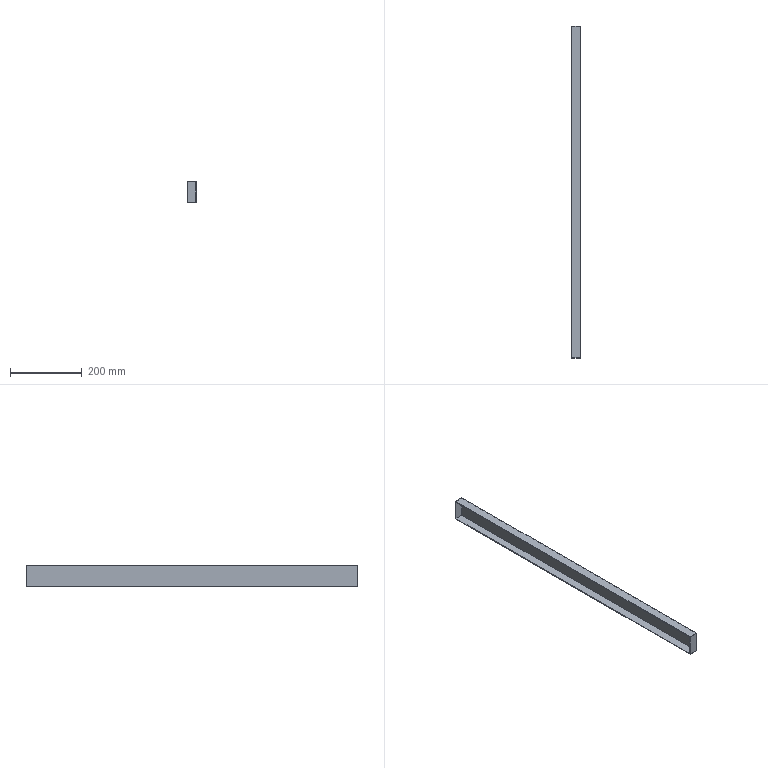Component | SolidWorks | SolderBox-1 | 1 solid | 11 faces | box 25 x 925 x 60 mm | volume 201252 mm3 | plane 11 | material Plain Carbon Steel
build123d program:
from build123d import *

# Parameters (mm, degrees)
SKETCH1_W           = 925
SKETCH1_H           = 60
BOSS_EXTRUDE1_DEPTH = 25
SHELL1_T            = -2


with BuildPart() as part:
    # Sketch1 → Boss-Extrude1 (new body)
    with BuildSketch(Plane.XY):
        Rectangle(SKETCH1_W, SKETCH1_H)
    extrude(amount=BOSS_EXTRUDE1_DEPTH)

    # Shell1
    shell1_openings = [part.faces().sort_by_distance(p)[0] for p in [
        (0, 0, 25),
    ]]
    offset(amount=SHELL1_T, openings=shell1_openings, kind=Kind.INTERSECTION)


solid = part.part

# Placed as in the assembly
solid = solid.moved(Location((-806.135, 72.093, 1073.102), (90, -90, 0)))
STEP:
#1=COLOUR_RGB('',0.7922,0.8196,0.9333);
#2=FILL_AREA_STYLE_COLOUR('',#1);
#3=FILL_AREA_STYLE('',(#2));
#4=SURFACE_STYLE_FILL_AREA(#3);
#5=SURFACE_SIDE_STYLE('',(#4));
#6=SURFACE_STYLE_USAGE(.BOTH.,#5);
#7=PRESENTATION_STYLE_ASSIGNMENT((#6));
#8=CARTESIAN_POINT('',(-31.738,21.047,43.429));
#9=VERTEX_POINT('',#8);
#10=CARTESIAN_POINT('',(-31.738,21.047,41.067));
#11=VERTEX_POINT('',#10);
#12=CARTESIAN_POINT('',(-31.738,21.047,41.067));
#13=DIRECTION('',(-0.,0.,-1.));
#14=VECTOR('',#13,39.37);
#15=LINE('',#12,#14);
#16=EDGE_CURVE('',#9,#11,#15,.T.);
#17=ORIENTED_EDGE('',*,*,#16,.T.);
#18=CARTESIAN_POINT('',(-32.722,21.047,41.067));
#19=VERTEX_POINT('',#18);
#20=CARTESIAN_POINT('',(-32.722,21.047,41.067));
#21=DIRECTION('',(1.,0.,-0.));
#22=VECTOR('',#21,39.37);
#23=LINE('',#20,#22);
#24=EDGE_CURVE('',#19,#11,#23,.T.);
#25=ORIENTED_EDGE('',*,*,#24,.F.);
#26=CARTESIAN_POINT('',(-32.722,21.047,43.429));
#27=VERTEX_POINT('',#26);
#28=CARTESIAN_POINT('',(-32.722,21.047,41.067));
#29=DIRECTION('',(-0.,0.,-1.));
#30=VECTOR('',#29,39.37);
#31=LINE('',#28,#30);
#32=EDGE_CURVE('',#27,#19,#31,.T.);
#33=ORIENTED_EDGE('',*,*,#32,.F.);
#34=CARTESIAN_POINT('',(-32.722,21.047,43.429));
#35=DIRECTION('',(1.,0.,-0.));
#36=VECTOR('',#35,39.37);
#37=LINE('',#34,#36);
#38=EDGE_CURVE('',#27,#9,#37,.T.);
#39=ORIENTED_EDGE('',*,*,#38,.T.);
#40=EDGE_LOOP('',(#17,#25,#33,#39));
#41=FACE_OUTER_BOUND('',#40,.T.);
#42=CARTESIAN_POINT('',(-32.722,21.047,41.067));
#43=DIRECTION('',(0.,-1.,-0.));
#44=DIRECTION('',(1.,0.,-0.));
#45=AXIS2_PLACEMENT_3D('',#42,#43,#44);
#46=PLANE('',#45);
#47=ADVANCED_FACE('',(#41),#46,.F.);
#48=CARTESIAN_POINT('',(-31.738,-15.37,41.067));
#49=VERTEX_POINT('',#48);
#50=CARTESIAN_POINT('',(-31.738,-15.37,41.067));
#51=DIRECTION('',(0.,-1.,0.));
#52=VECTOR('',#51,39.37);
#53=LINE('',#50,#52);
#54=EDGE_CURVE('',#11,#49,#53,.T.);
#55=ORIENTED_EDGE('',*,*,#54,.T.);
#56=CARTESIAN_POINT('',(-32.722,-15.37,41.067));
#57=VERTEX_POINT('',#56);
#58=CARTESIAN_POINT('',(-32.722,-15.37,41.067));
#59=DIRECTION('',(1.,0.,-0.));
#60=VECTOR('',#59,39.37);
#61=LINE('',#58,#60);
#62=EDGE_CURVE('',#57,#49,#61,.T.);
#63=ORIENTED_EDGE('',*,*,#62,.F.);
#64=CARTESIAN_POINT('',(-32.722,-15.37,41.067));
#65=DIRECTION('',(0.,-1.,0.));
#66=VECTOR('',#65,39.37);
#67=LINE('',#64,#66);
#68=EDGE_CURVE('',#19,#57,#67,.T.);
#69=ORIENTED_EDGE('',*,*,#68,.F.);
#70=ORIENTED_EDGE('',*,*,#24,.T.);
#71=EDGE_LOOP('',(#55,#63,#69,#70));
#72=FACE_OUTER_BOUND('',#71,.T.);
#73=CARTESIAN_POINT('',(-32.722,-15.37,41.067));
#74=DIRECTION('',(0.,0.,1.));
#75=DIRECTION('',(-0.,1.,-0.));
#76=AXIS2_PLACEMENT_3D('',#73,#74,#75);
#77=PLANE('',#76);
#78=ADVANCED_FACE('',(#72),#77,.F.);
#79=CARTESIAN_POINT('',(-31.738,-15.37,43.429));
#80=VERTEX_POINT('',#79);
#81=CARTESIAN_POINT('',(-31.738,-15.37,41.067));
#82=DIRECTION('',(0.,-0.,1.));
#83=VECTOR('',#82,39.37);
#84=LINE('',#81,#83);
#85=EDGE_CURVE('',#49,#80,#84,.T.);
#86=ORIENTED_EDGE('',*,*,#85,.T.);
#87=CARTESIAN_POINT('',(-32.722,-15.37,43.429));
#88=VERTEX_POINT('',#87);
#89=CARTESIAN_POINT('',(-32.722,-15.37,43.429));
#90=DIRECTION('',(1.,0.,-0.));
#91=VECTOR('',#90,39.37);
#92=LINE('',#89,#91);
#93=EDGE_CURVE('',#88,#80,#92,.T.);
#94=ORIENTED_EDGE('',*,*,#93,.F.);
#95=CARTESIAN_POINT('',(-32.722,-15.37,41.067));
#96=DIRECTION('',(0.,-0.,1.));
#97=VECTOR('',#96,39.37);
#98=LINE('',#95,#97);
#99=EDGE_CURVE('',#57,#88,#98,.T.);
#100=ORIENTED_EDGE('',*,*,#99,.F.);
#101=ORIENTED_EDGE('',*,*,#62,.T.);
#102=EDGE_LOOP('',(#86,#94,#100,#101));
#103=FACE_OUTER_BOUND('',#102,.T.);
#104=CARTESIAN_POINT('',(-32.722,-15.37,41.067));
#105=DIRECTION('',(-0.,1.,0.));
#106=DIRECTION('',(-1.,-0.,0.));
#107=AXIS2_PLACEMENT_3D('',#104,#105,#106);
#108=PLANE('',#107);
#109=ADVANCED_FACE('',(#103),#108,.F.);
#110=CARTESIAN_POINT('',(-31.738,-15.37,43.429));
#111=DIRECTION('',(-0.,1.,-0.));
#112=VECTOR('',#111,39.37);
#113=LINE('',#110,#112);
#114=EDGE_CURVE('',#80,#9,#113,.T.);
#115=ORIENTED_EDGE('',*,*,#114,.T.);
#116=ORIENTED_EDGE('',*,*,#38,.F.);
#117=CARTESIAN_POINT('',(-32.722,-15.37,43.429));
#118=DIRECTION('',(-0.,1.,-0.));
#119=VECTOR('',#118,39.37);
#120=LINE('',#117,#119);
#121=EDGE_CURVE('',#88,#27,#120,.T.);
#122=ORIENTED_EDGE('',*,*,#121,.F.);
#123=ORIENTED_EDGE('',*,*,#93,.T.);
#124=EDGE_LOOP('',(#115,#116,#122,#123));
#125=FACE_OUTER_BOUND('',#124,.T.);
#126=CARTESIAN_POINT('',(-32.722,-15.37,43.429));
#127=DIRECTION('',(-0.,-0.,-1.));
#128=DIRECTION('',(0.,-1.,0.));
#129=AXIS2_PLACEMENT_3D('',#126,#127,#128);
#130=PLANE('',#129);
#131=ADVANCED_FACE('',(#125),#130,.F.);
#132=CARTESIAN_POINT('',(-32.722,20.968,43.35));
#133=VERTEX_POINT('',#132);
#134=CARTESIAN_POINT('',(-32.722,20.968,41.146));
#135=VERTEX_POINT('',#134);
#136=CARTESIAN_POINT('',(-32.722,20.968,41.067));
#137=DIRECTION('',(-0.,0.,-1.));
#138=VECTOR('',#137,39.37);
#139=LINE('',#136,#138);
#140=EDGE_CURVE('',#133,#135,#139,.T.);
#141=ORIENTED_EDGE('',*,*,#140,.F.);
#142=CARTESIAN_POINT('',(-32.722,-15.292,43.35));
#143=VERTEX_POINT('',#142);
#144=CARTESIAN_POINT('',(-32.722,-15.37,43.35));
#145=DIRECTION('',(-0.,1.,-0.));
#146=VECTOR('',#145,39.37);
#147=LINE('',#144,#146);
#148=EDGE_CURVE('',#143,#133,#147,.T.);
#149=ORIENTED_EDGE('',*,*,#148,.F.);
#150=CARTESIAN_POINT('',(-32.722,-15.292,41.146));
#151=VERTEX_POINT('',#150);
#152=CARTESIAN_POINT('',(-32.722,-15.292,41.067));
#153=DIRECTION('',(0.,-0.,1.));
#154=VECTOR('',#153,39.37);
#155=LINE('',#152,#154);
#156=EDGE_CURVE('',#151,#143,#155,.T.);
#157=ORIENTED_EDGE('',*,*,#156,.F.);
#158=CARTESIAN_POINT('',(-32.722,-15.37,41.146));
#159=DIRECTION('',(0.,-1.,0.));
#160=VECTOR('',#159,39.37);
#161=LINE('',#158,#160);
#162=EDGE_CURVE('',#135,#151,#161,.T.);
#163=ORIENTED_EDGE('',*,*,#162,.F.);
#164=EDGE_LOOP('',(#141,#149,#157,#163));
#165=FACE_BOUND('',#164,.T.);
#166=ORIENTED_EDGE('',*,*,#32,.T.);
#167=ORIENTED_EDGE('',*,*,#68,.T.);
#168=ORIENTED_EDGE('',*,*,#99,.T.);
#169=ORIENTED_EDGE('',*,*,#121,.T.);
#170=EDGE_LOOP('',(#166,#167,#168,#169));
#171=FACE_OUTER_BOUND('',#170,.T.);
#172=CARTESIAN_POINT('',(-32.722,2.838,42.248));
#173=DIRECTION('',(-1.,-0.,0.));
#174=DIRECTION('',(0.,-1.,-0.));
#175=AXIS2_PLACEMENT_3D('',#172,#173,#174);
#176=PLANE('',#175);
#177=ADVANCED_FACE('',(#165,#171),#176,.T.);
#178=ORIENTED_EDGE('',*,*,#16,.F.);
#179=ORIENTED_EDGE('',*,*,#114,.F.);
#180=ORIENTED_EDGE('',*,*,#85,.F.);
#181=ORIENTED_EDGE('',*,*,#54,.F.);
#182=EDGE_LOOP('',(#178,#179,#180,#181));
#183=FACE_OUTER_BOUND('',#182,.T.);
#184=CARTESIAN_POINT('',(-31.738,2.838,42.248));
#185=DIRECTION('',(-1.,-0.,0.));
#186=DIRECTION('',(0.,-1.,-0.));
#187=AXIS2_PLACEMENT_3D('',#184,#185,#186);
#188=PLANE('',#187);
#189=ADVANCED_FACE('',(#183),#188,.F.);
#190=CARTESIAN_POINT('',(-31.816,20.968,43.35));
#191=VERTEX_POINT('',#190);
#192=CARTESIAN_POINT('',(-31.816,20.968,41.146));
#193=VERTEX_POINT('',#192);
#194=CARTESIAN_POINT('',(-31.816,20.968,41.067));
#195=DIRECTION('',(-0.,0.,-1.));
#196=VECTOR('',#195,39.37);
#197=LINE('',#194,#196);
#198=EDGE_CURVE('',#191,#193,#197,.T.);
#199=ORIENTED_EDGE('',*,*,#198,.F.);
#200=CARTESIAN_POINT('',(-32.722,20.968,43.35));
#201=DIRECTION('',(1.,0.,-0.));
#202=VECTOR('',#201,39.37);
#203=LINE('',#200,#202);
#204=EDGE_CURVE('',#133,#191,#203,.T.);
#205=ORIENTED_EDGE('',*,*,#204,.F.);
#206=ORIENTED_EDGE('',*,*,#140,.T.);
#207=CARTESIAN_POINT('',(-32.722,20.968,41.146));
#208=DIRECTION('',(1.,0.,-0.));
#209=VECTOR('',#208,39.37);
#210=LINE('',#207,#209);
#211=EDGE_CURVE('',#135,#193,#210,.T.);
#212=ORIENTED_EDGE('',*,*,#211,.T.);
#213=EDGE_LOOP('',(#199,#205,#206,#212));
#214=FACE_OUTER_BOUND('',#213,.T.);
#215=CARTESIAN_POINT('',(-32.722,20.968,41.067));
#216=DIRECTION('',(0.,-1.,-0.));
#217=DIRECTION('',(1.,0.,-0.));
#218=AXIS2_PLACEMENT_3D('',#215,#216,#217);
#219=PLANE('',#218);
#220=ADVANCED_FACE('',(#214),#219,.T.);
#221=CARTESIAN_POINT('',(-31.816,-15.292,41.146));
#222=VERTEX_POINT('',#221);
#223=CARTESIAN_POINT('',(-31.816,-15.37,41.146));
#224=DIRECTION('',(0.,-1.,0.));
#225=VECTOR('',#224,39.37);
#226=LINE('',#223,#225);
#227=EDGE_CURVE('',#193,#222,#226,.T.);
#228=ORIENTED_EDGE('',*,*,#227,.F.);
#229=ORIENTED_EDGE('',*,*,#211,.F.);
#230=ORIENTED_EDGE('',*,*,#162,.T.);
#231=CARTESIAN_POINT('',(-32.722,-15.292,41.146));
#232=DIRECTION('',(1.,0.,-0.));
#233=VECTOR('',#232,39.37);
#234=LINE('',#231,#233);
#235=EDGE_CURVE('',#151,#222,#234,.T.);
#236=ORIENTED_EDGE('',*,*,#235,.T.);
#237=EDGE_LOOP('',(#228,#229,#230,#236));
#238=FACE_OUTER_BOUND('',#237,.T.);
#239=CARTESIAN_POINT('',(-32.722,-15.37,41.146));
#240=DIRECTION('',(0.,0.,1.));
#241=DIRECTION('',(-0.,1.,-0.));
#242=AXIS2_PLACEMENT_3D('',#239,#240,#241);
#243=PLANE('',#242);
#244=ADVANCED_FACE('',(#238),#243,.T.);
#245=CARTESIAN_POINT('',(-31.816,-15.292,43.35));
#246=VERTEX_POINT('',#245);
#247=CARTESIAN_POINT('',(-31.816,-15.292,41.067));
#248=DIRECTION('',(0.,-0.,1.));
#249=VECTOR('',#248,39.37);
#250=LINE('',#247,#249);
#251=EDGE_CURVE('',#222,#246,#250,.T.);
#252=ORIENTED_EDGE('',*,*,#251,.F.);
#253=ORIENTED_EDGE('',*,*,#235,.F.);
#254=ORIENTED_EDGE('',*,*,#156,.T.);
#255=CARTESIAN_POINT('',(-32.722,-15.292,43.35));
#256=DIRECTION('',(1.,0.,-0.));
#257=VECTOR('',#256,39.37);
#258=LINE('',#255,#257);
#259=EDGE_CURVE('',#143,#246,#258,.T.);
#260=ORIENTED_EDGE('',*,*,#259,.T.);
#261=EDGE_LOOP('',(#252,#253,#254,#260));
#262=FACE_OUTER_BOUND('',#261,.T.);
#263=CARTESIAN_POINT('',(-32.722,-15.292,41.067));
#264=DIRECTION('',(-0.,1.,0.));
#265=DIRECTION('',(-1.,-0.,0.));
#266=AXIS2_PLACEMENT_3D('',#263,#264,#265);
#267=PLANE('',#266);
#268=ADVANCED_FACE('',(#262),#267,.T.);
#269=CARTESIAN_POINT('',(-31.816,-15.37,43.35));
#270=DIRECTION('',(-0.,1.,-0.));
#271=VECTOR('',#270,39.37);
#272=LINE('',#269,#271);
#273=EDGE_CURVE('',#246,#191,#272,.T.);
#274=ORIENTED_EDGE('',*,*,#273,.F.);
#275=ORIENTED_EDGE('',*,*,#259,.F.);
#276=ORIENTED_EDGE('',*,*,#148,.T.);
#277=ORIENTED_EDGE('',*,*,#204,.T.);
#278=EDGE_LOOP('',(#274,#275,#276,#277));
#279=FACE_OUTER_BOUND('',#278,.T.);
#280=CARTESIAN_POINT('',(-32.722,-15.37,43.35));
#281=DIRECTION('',(-0.,-0.,-1.));
#282=DIRECTION('',(0.,-1.,0.));
#283=AXIS2_PLACEMENT_3D('',#280,#281,#282);
#284=PLANE('',#283);
#285=ADVANCED_FACE('',(#279),#284,.T.);
#286=ORIENTED_EDGE('',*,*,#198,.T.);
#287=ORIENTED_EDGE('',*,*,#227,.T.);
#288=ORIENTED_EDGE('',*,*,#251,.T.);
#289=ORIENTED_EDGE('',*,*,#273,.T.);
#290=EDGE_LOOP('',(#286,#287,#288,#289));
#291=FACE_OUTER_BOUND('',#290,.T.);
#292=CARTESIAN_POINT('',(-31.816,2.838,42.248));
#293=DIRECTION('',(-1.,-0.,0.));
#294=DIRECTION('',(0.,-1.,-0.));
#295=AXIS2_PLACEMENT_3D('',#292,#293,#294);
#296=PLANE('',#295);
#297=ADVANCED_FACE('',(#291),#296,.T.);
#298=CLOSED_SHELL('',(#47,#78,#109,#131,#177,#189,#220,#244,#268,#285,#297));
#299=MANIFOLD_SOLID_BREP('',#298);
#300=STYLED_ITEM('',(#7),#299);
#301=PRESENTATION_LAYER_ASSIGNMENT('','',(#300));
#302=CARTESIAN_POINT('',(0.,0.,0.));
#303=DIRECTION('',(0.,0.,1.));
#304=DIRECTION('',(1.,0.,0.));
#305=AXIS2_PLACEMENT_3D('',#302,#303,#304);
#306=(LENGTH_UNIT()NAMED_UNIT(*)SI_UNIT($,.METRE.));
#307=LENGTH_MEASURE_WITH_UNIT(LENGTH_MEASURE(0.0254),#306);
#308=DIMENSIONAL_EXPONENTS(1.,0.,0.,0.,0.,0.,0.);
#309=(CONVERSION_BASED_UNIT('',#307)LENGTH_UNIT()NAMED_UNIT(#308));
#310=UNCERTAINTY_MEASURE_WITH_UNIT(LENGTH_MEASURE(0.00001),#309,'','');
#311=(NAMED_UNIT(*)PLANE_ANGLE_UNIT()SI_UNIT($,.RADIAN.));
#312=(NAMED_UNIT(*)SI_UNIT($,.STERADIAN.)SOLID_ANGLE_UNIT());
#313=(GEOMETRIC_REPRESENTATION_CONTEXT(3)GLOBAL_UNCERTAINTY_ASSIGNED_CONTEXT((#310))GLOBAL_UNIT_ASSIGNED_CONTEXT((#309,#311,#312))REPRESENTATION_CONTEXT('',''));
#314=ADVANCED_BREP_SHAPE_REPRESENTATION('',(#299,#305),#313);
#315=(LENGTH_UNIT()NAMED_UNIT(*)SI_UNIT($,.METRE.));
#316=LENGTH_MEASURE_WITH_UNIT(LENGTH_MEASURE(0.0254),#315);
#317=DIMENSIONAL_EXPONENTS(1.,0.,0.,0.,0.,0.,0.);
#318=(CONVERSION_BASED_UNIT('',#316)LENGTH_UNIT()NAMED_UNIT(#317));
#319=UNCERTAINTY_MEASURE_WITH_UNIT(LENGTH_MEASURE(0.00001),#318,'','');
#320=(NAMED_UNIT(*)PLANE_ANGLE_UNIT()SI_UNIT($,.RADIAN.));
#321=(NAMED_UNIT(*)SI_UNIT($,.STERADIAN.)SOLID_ANGLE_UNIT());
#322=(GEOMETRIC_REPRESENTATION_CONTEXT(3)GLOBAL_UNCERTAINTY_ASSIGNED_CONTEXT((#319))GLOBAL_UNIT_ASSIGNED_CONTEXT((#318,#320,#321))REPRESENTATION_CONTEXT('',''));
#323=MECHANICAL_DESIGN_GEOMETRIC_PRESENTATION_REPRESENTATION('',(#300),#322);